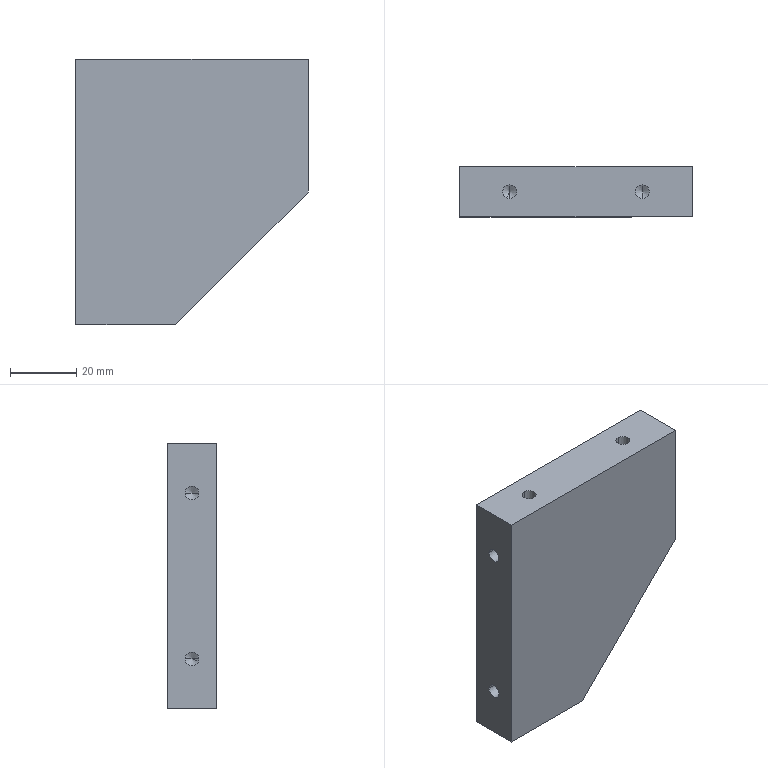Component | SolidWorks | BeveledAluminumSupport-1 | 1 solid | 23 faces | box 70 x 15 x 80 mm | volume 71290 mm3 | cylinder 8 | cone 8 | plane 7 | commonest cylinder face diameters 4.2 x8
build123d program:
from build123d import *

# Parameters (mm, degrees)
BOSS_EXTRUDE1_DEPTH   = 7.5
M5_TAPPED_HOLE1_D     = 4.2
M5_TAPPED_HOLE1_DEPTH = 12.4
M5_TAPPED_HOLE1_TIP   = 1.212
M5_TAPPED_HOLE2_D     = 4.2
M5_TAPPED_HOLE2_DEPTH = 12.4
M5_TAPPED_HOLE2_TIP   = 1.212


with BuildPart() as part:
    # Sketch1 → Boss-Extrude1 (new, symmetric)
    with BuildSketch(Plane.XY):
        Polygon((30, 80), (70, 40), (70, 0), (0, 0), (0, 80), align=None)
    extrude(amount=BOSS_EXTRUDE1_DEPTH, both=True)

    # M5 Tapped Hole1
    with Locations(Plane(origin=(0, 65, 0), x_dir=(0, 0, -1), z_dir=(-1, 0, 0))):
        with Locations((0, 0), (0, 50)):
            Hole(M5_TAPPED_HOLE1_D / 2, depth=M5_TAPPED_HOLE1_DEPTH)
            with Locations((0, 0, -(M5_TAPPED_HOLE1_DEPTH + M5_TAPPED_HOLE1_TIP / 2))):  # 120° drill point
                Cone(0, M5_TAPPED_HOLE1_D / 2, M5_TAPPED_HOLE1_TIP, mode=Mode.SUBTRACT)

    # M5 Tapped Hole2
    with Locations(Plane(origin=(15, 0, 0), x_dir=(0, 0, -1), z_dir=(0, -1, 0))):
        with Locations((0, 0), (0, 40)):
            Hole(M5_TAPPED_HOLE2_D / 2, depth=M5_TAPPED_HOLE2_DEPTH)
            with Locations((0, 0, -(M5_TAPPED_HOLE2_DEPTH + M5_TAPPED_HOLE2_TIP / 2))):  # 120° drill point
                Cone(0, M5_TAPPED_HOLE2_D / 2, M5_TAPPED_HOLE2_TIP, mode=Mode.SUBTRACT)


solid = part.part

# Placed as in the assembly
solid = solid.moved(Location((2.915, 37.185, 71.225), (-90, 0, 0)))
STEP:
#1=COLOUR_RGB('',0.7922,0.8196,0.9333);
#2=FILL_AREA_STYLE_COLOUR('',#1);
#3=FILL_AREA_STYLE('',(#2));
#4=SURFACE_STYLE_FILL_AREA(#3);
#5=SURFACE_SIDE_STYLE('',(#4));
#6=SURFACE_STYLE_USAGE(.BOTH.,#5);
#7=PRESENTATION_STYLE_ASSIGNMENT((#6));
#8=CARTESIAN_POINT('',(0.7053,1.547,2.316));
#9=VERTEX_POINT('',#8);
#10=CARTESIAN_POINT('',(0.7053,1.381,2.316));
#11=VERTEX_POINT('',#10);
#12=CARTESIAN_POINT('',(0.7053,1.464,2.316));
#13=DIRECTION('',(0.,0.,1.));
#14=DIRECTION('',(0.,-1.,0.));
#15=AXIS2_PLACEMENT_3D('',#12,#13,#14);
#16=CIRCLE('',#15,0.08268);
#17=EDGE_CURVE('',#9,#11,#16,.T.);
#18=ORIENTED_EDGE('',*,*,#17,.F.);
#19=CARTESIAN_POINT('',(0.7053,1.547,2.804));
#20=VERTEX_POINT('',#19);
#21=CARTESIAN_POINT('',(0.7053,1.547,2.804));
#22=DIRECTION('',(0.,0.,1.));
#23=VECTOR('',#22,39.37);
#24=LINE('',#21,#23);
#25=EDGE_CURVE('',#9,#20,#24,.T.);
#26=ORIENTED_EDGE('',*,*,#25,.T.);
#27=CARTESIAN_POINT('',(0.7053,1.381,2.804));
#28=VERTEX_POINT('',#27);
#29=CARTESIAN_POINT('',(0.7053,1.464,2.804));
#30=DIRECTION('',(0.,0.,1.));
#31=DIRECTION('',(0.,-1.,0.));
#32=AXIS2_PLACEMENT_3D('',#29,#30,#31);
#33=CIRCLE('',#32,0.08268);
#34=EDGE_CURVE('',#20,#28,#33,.T.);
#35=ORIENTED_EDGE('',*,*,#34,.T.);
#36=CARTESIAN_POINT('',(0.7053,1.381,2.804));
#37=DIRECTION('',(0.,0.,1.));
#38=VECTOR('',#37,39.37);
#39=LINE('',#36,#38);
#40=EDGE_CURVE('',#11,#28,#39,.T.);
#41=ORIENTED_EDGE('',*,*,#40,.F.);
#42=EDGE_LOOP('',(#18,#26,#35,#41));
#43=FACE_OUTER_BOUND('',#42,.T.);
#44=CARTESIAN_POINT('',(0.7053,1.464,2.804));
#45=DIRECTION('',(0.,0.,1.));
#46=DIRECTION('',(0.,-1.,0.));
#47=AXIS2_PLACEMENT_3D('',#44,#45,#46);
#48=CYLINDRICAL_SURFACE('',#47,0.08268);
#49=ADVANCED_FACE('',(#43),#48,.F.);
#50=CARTESIAN_POINT('',(0.7053,1.464,2.268));
#51=VERTEX_POINT('',#50);
#52=CARTESIAN_POINT('',(0.7053,1.381,2.316));
#53=DIRECTION('',(0.,-0.866,0.5));
#54=VECTOR('',#53,39.37);
#55=LINE('',#52,#54);
#56=EDGE_CURVE('',#51,#11,#55,.T.);
#57=ORIENTED_EDGE('',*,*,#56,.F.);
#58=CARTESIAN_POINT('',(0.7053,1.547,2.316));
#59=DIRECTION('',(0.,0.866,0.5));
#60=VECTOR('',#59,39.37);
#61=LINE('',#58,#60);
#62=EDGE_CURVE('',#51,#9,#61,.T.);
#63=ORIENTED_EDGE('',*,*,#62,.T.);
#64=ORIENTED_EDGE('',*,*,#17,.T.);
#65=EDGE_LOOP('',(#57,#63,#64));
#66=FACE_OUTER_BOUND('',#65,.T.);
#67=CARTESIAN_POINT('',(0.7053,1.464,2.316));
#68=DIRECTION('',(0.,0.,1.));
#69=DIRECTION('',(0.,-1.,0.));
#70=AXIS2_PLACEMENT_3D('',#67,#68,#69);
#71=CONICAL_SURFACE('',#70,0.08268,1.047);
#72=ADVANCED_FACE('',(#66),#71,.F.);
#73=CARTESIAN_POINT('',(2.28,1.547,2.316));
#74=VERTEX_POINT('',#73);
#75=CARTESIAN_POINT('',(2.28,1.381,2.316));
#76=VERTEX_POINT('',#75);
#77=CARTESIAN_POINT('',(2.28,1.464,2.316));
#78=DIRECTION('',(0.,0.,1.));
#79=DIRECTION('',(0.,-1.,0.));
#80=AXIS2_PLACEMENT_3D('',#77,#78,#79);
#81=CIRCLE('',#80,0.08268);
#82=EDGE_CURVE('',#74,#76,#81,.T.);
#83=ORIENTED_EDGE('',*,*,#82,.F.);
#84=CARTESIAN_POINT('',(2.28,1.547,2.804));
#85=VERTEX_POINT('',#84);
#86=CARTESIAN_POINT('',(2.28,1.547,2.804));
#87=DIRECTION('',(0.,0.,1.));
#88=VECTOR('',#87,39.37);
#89=LINE('',#86,#88);
#90=EDGE_CURVE('',#74,#85,#89,.T.);
#91=ORIENTED_EDGE('',*,*,#90,.T.);
#92=CARTESIAN_POINT('',(2.28,1.381,2.804));
#93=VERTEX_POINT('',#92);
#94=CARTESIAN_POINT('',(2.28,1.464,2.804));
#95=DIRECTION('',(0.,0.,1.));
#96=DIRECTION('',(0.,-1.,0.));
#97=AXIS2_PLACEMENT_3D('',#94,#95,#96);
#98=CIRCLE('',#97,0.08268);
#99=EDGE_CURVE('',#85,#93,#98,.T.);
#100=ORIENTED_EDGE('',*,*,#99,.T.);
#101=CARTESIAN_POINT('',(2.28,1.381,2.804));
#102=DIRECTION('',(0.,0.,1.));
#103=VECTOR('',#102,39.37);
#104=LINE('',#101,#103);
#105=EDGE_CURVE('',#76,#93,#104,.T.);
#106=ORIENTED_EDGE('',*,*,#105,.F.);
#107=EDGE_LOOP('',(#83,#91,#100,#106));
#108=FACE_OUTER_BOUND('',#107,.T.);
#109=CARTESIAN_POINT('',(2.28,1.464,2.804));
#110=DIRECTION('',(0.,0.,1.));
#111=DIRECTION('',(0.,-1.,0.));
#112=AXIS2_PLACEMENT_3D('',#109,#110,#111);
#113=CYLINDRICAL_SURFACE('',#112,0.08268);
#114=ADVANCED_FACE('',(#108),#113,.F.);
#115=CARTESIAN_POINT('',(2.28,1.464,2.268));
#116=VERTEX_POINT('',#115);
#117=CARTESIAN_POINT('',(2.28,1.381,2.316));
#118=DIRECTION('',(0.,-0.866,0.5));
#119=VECTOR('',#118,39.37);
#120=LINE('',#117,#119);
#121=EDGE_CURVE('',#116,#76,#120,.T.);
#122=ORIENTED_EDGE('',*,*,#121,.F.);
#123=CARTESIAN_POINT('',(2.28,1.547,2.316));
#124=DIRECTION('',(0.,0.866,0.5));
#125=VECTOR('',#124,39.37);
#126=LINE('',#123,#125);
#127=EDGE_CURVE('',#116,#74,#126,.T.);
#128=ORIENTED_EDGE('',*,*,#127,.T.);
#129=ORIENTED_EDGE('',*,*,#82,.T.);
#130=EDGE_LOOP('',(#122,#128,#129));
#131=FACE_OUTER_BOUND('',#130,.T.);
#132=CARTESIAN_POINT('',(2.28,1.464,2.316));
#133=DIRECTION('',(0.,0.,1.));
#134=DIRECTION('',(0.,-1.,0.));
#135=AXIS2_PLACEMENT_3D('',#132,#133,#134);
#136=CONICAL_SURFACE('',#135,0.08268,1.047);
#137=ADVANCED_FACE('',(#131),#136,.F.);
#138=CARTESIAN_POINT('',(0.603,1.381,0.2451));
#139=VERTEX_POINT('',#138);
#140=CARTESIAN_POINT('',(0.603,1.547,0.2451));
#141=VERTEX_POINT('',#140);
#142=CARTESIAN_POINT('',(0.603,1.464,0.2451));
#143=DIRECTION('',(-1.,0.,0.));
#144=DIRECTION('',(0.,1.,0.));
#145=AXIS2_PLACEMENT_3D('',#142,#143,#144);
#146=CIRCLE('',#145,0.08268);
#147=EDGE_CURVE('',#139,#141,#146,.T.);
#148=ORIENTED_EDGE('',*,*,#147,.F.);
#149=CARTESIAN_POINT('',(0.1148,1.381,0.2451));
#150=VERTEX_POINT('',#149);
#151=CARTESIAN_POINT('',(0.1148,1.381,0.2451));
#152=DIRECTION('',(-1.,0.,0.));
#153=VECTOR('',#152,39.37);
#154=LINE('',#151,#153);
#155=EDGE_CURVE('',#139,#150,#154,.T.);
#156=ORIENTED_EDGE('',*,*,#155,.T.);
#157=CARTESIAN_POINT('',(0.1148,1.547,0.2451));
#158=VERTEX_POINT('',#157);
#159=CARTESIAN_POINT('',(0.1148,1.464,0.2451));
#160=DIRECTION('',(-1.,0.,0.));
#161=DIRECTION('',(0.,1.,0.));
#162=AXIS2_PLACEMENT_3D('',#159,#160,#161);
#163=CIRCLE('',#162,0.08268);
#164=EDGE_CURVE('',#150,#158,#163,.T.);
#165=ORIENTED_EDGE('',*,*,#164,.T.);
#166=CARTESIAN_POINT('',(0.1148,1.547,0.2451));
#167=DIRECTION('',(-1.,0.,0.));
#168=VECTOR('',#167,39.37);
#169=LINE('',#166,#168);
#170=EDGE_CURVE('',#141,#158,#169,.T.);
#171=ORIENTED_EDGE('',*,*,#170,.F.);
#172=EDGE_LOOP('',(#148,#156,#165,#171));
#173=FACE_OUTER_BOUND('',#172,.T.);
#174=CARTESIAN_POINT('',(0.1148,1.464,0.2451));
#175=DIRECTION('',(-1.,0.,0.));
#176=DIRECTION('',(0.,1.,0.));
#177=AXIS2_PLACEMENT_3D('',#174,#175,#176);
#178=CYLINDRICAL_SURFACE('',#177,0.08268);
#179=ADVANCED_FACE('',(#173),#178,.F.);
#180=CARTESIAN_POINT('',(0.6507,1.464,0.2451));
#181=VERTEX_POINT('',#180);
#182=CARTESIAN_POINT('',(0.603,1.547,0.2451));
#183=DIRECTION('',(-0.5,0.866,0.));
#184=VECTOR('',#183,39.37);
#185=LINE('',#182,#184);
#186=EDGE_CURVE('',#181,#141,#185,.T.);
#187=ORIENTED_EDGE('',*,*,#186,.F.);
#188=CARTESIAN_POINT('',(0.603,1.381,0.2451));
#189=DIRECTION('',(-0.5,-0.866,-0.));
#190=VECTOR('',#189,39.37);
#191=LINE('',#188,#190);
#192=EDGE_CURVE('',#181,#139,#191,.T.);
#193=ORIENTED_EDGE('',*,*,#192,.T.);
#194=ORIENTED_EDGE('',*,*,#147,.T.);
#195=EDGE_LOOP('',(#187,#193,#194));
#196=FACE_OUTER_BOUND('',#195,.T.);
#197=CARTESIAN_POINT('',(0.603,1.464,0.2451));
#198=DIRECTION('',(-1.,0.,0.));
#199=DIRECTION('',(0.,1.,0.));
#200=AXIS2_PLACEMENT_3D('',#197,#198,#199);
#201=CONICAL_SURFACE('',#200,0.08268,1.047);
#202=ADVANCED_FACE('',(#196),#201,.F.);
#203=CARTESIAN_POINT('',(0.603,1.381,2.214));
#204=VERTEX_POINT('',#203);
#205=CARTESIAN_POINT('',(0.603,1.547,2.214));
#206=VERTEX_POINT('',#205);
#207=CARTESIAN_POINT('',(0.603,1.464,2.214));
#208=DIRECTION('',(-1.,0.,0.));
#209=DIRECTION('',(0.,1.,0.));
#210=AXIS2_PLACEMENT_3D('',#207,#208,#209);
#211=CIRCLE('',#210,0.08268);
#212=EDGE_CURVE('',#204,#206,#211,.T.);
#213=ORIENTED_EDGE('',*,*,#212,.F.);
#214=CARTESIAN_POINT('',(0.1148,1.381,2.214));
#215=VERTEX_POINT('',#214);
#216=CARTESIAN_POINT('',(0.1148,1.381,2.214));
#217=DIRECTION('',(-1.,0.,0.));
#218=VECTOR('',#217,39.37);
#219=LINE('',#216,#218);
#220=EDGE_CURVE('',#204,#215,#219,.T.);
#221=ORIENTED_EDGE('',*,*,#220,.T.);
#222=CARTESIAN_POINT('',(0.1148,1.547,2.214));
#223=VERTEX_POINT('',#222);
#224=CARTESIAN_POINT('',(0.1148,1.464,2.214));
#225=DIRECTION('',(-1.,0.,0.));
#226=DIRECTION('',(0.,1.,0.));
#227=AXIS2_PLACEMENT_3D('',#224,#225,#226);
#228=CIRCLE('',#227,0.08268);
#229=EDGE_CURVE('',#215,#223,#228,.T.);
#230=ORIENTED_EDGE('',*,*,#229,.T.);
#231=CARTESIAN_POINT('',(0.1148,1.547,2.214));
#232=DIRECTION('',(-1.,0.,0.));
#233=VECTOR('',#232,39.37);
#234=LINE('',#231,#233);
#235=EDGE_CURVE('',#206,#223,#234,.T.);
#236=ORIENTED_EDGE('',*,*,#235,.F.);
#237=EDGE_LOOP('',(#213,#221,#230,#236));
#238=FACE_OUTER_BOUND('',#237,.T.);
#239=CARTESIAN_POINT('',(0.1148,1.464,2.214));
#240=DIRECTION('',(-1.,0.,0.));
#241=DIRECTION('',(0.,1.,0.));
#242=AXIS2_PLACEMENT_3D('',#239,#240,#241);
#243=CYLINDRICAL_SURFACE('',#242,0.08268);
#244=ADVANCED_FACE('',(#238),#243,.F.);
#245=CARTESIAN_POINT('',(0.6507,1.464,2.214));
#246=VERTEX_POINT('',#245);
#247=CARTESIAN_POINT('',(0.603,1.547,2.214));
#248=DIRECTION('',(-0.5,0.866,0.));
#249=VECTOR('',#248,39.37);
#250=LINE('',#247,#249);
#251=EDGE_CURVE('',#246,#206,#250,.T.);
#252=ORIENTED_EDGE('',*,*,#251,.F.);
#253=CARTESIAN_POINT('',(0.603,1.381,2.214));
#254=DIRECTION('',(-0.5,-0.866,-0.));
#255=VECTOR('',#254,39.37);
#256=LINE('',#253,#255);
#257=EDGE_CURVE('',#246,#204,#256,.T.);
#258=ORIENTED_EDGE('',*,*,#257,.T.);
#259=ORIENTED_EDGE('',*,*,#212,.T.);
#260=EDGE_LOOP('',(#252,#258,#259));
#261=FACE_OUTER_BOUND('',#260,.T.);
#262=CARTESIAN_POINT('',(0.603,1.464,2.214));
#263=DIRECTION('',(-1.,0.,0.));
#264=DIRECTION('',(0.,1.,0.));
#265=AXIS2_PLACEMENT_3D('',#262,#263,#264);
#266=CONICAL_SURFACE('',#265,0.08268,1.047);
#267=ADVANCED_FACE('',(#261),#266,.F.);
#268=CARTESIAN_POINT('',(0.1148,1.464,0.2451));
#269=DIRECTION('',(-1.,0.,0.));
#270=DIRECTION('',(0.,1.,0.));
#271=AXIS2_PLACEMENT_3D('',#268,#269,#270);
#272=CIRCLE('',#271,0.08268);
#273=EDGE_CURVE('',#158,#150,#272,.T.);
#274=ORIENTED_EDGE('',*,*,#273,.F.);
#275=ORIENTED_EDGE('',*,*,#164,.F.);
#276=EDGE_LOOP('',(#274,#275));
#277=FACE_BOUND('',#276,.T.);
#278=CARTESIAN_POINT('',(0.1148,1.464,2.214));
#279=DIRECTION('',(-1.,0.,0.));
#280=DIRECTION('',(0.,1.,0.));
#281=AXIS2_PLACEMENT_3D('',#278,#279,#280);
#282=CIRCLE('',#281,0.08268);
#283=EDGE_CURVE('',#223,#215,#282,.T.);
#284=ORIENTED_EDGE('',*,*,#283,.F.);
#285=ORIENTED_EDGE('',*,*,#229,.F.);
#286=EDGE_LOOP('',(#284,#285));
#287=FACE_BOUND('',#286,.T.);
#288=CARTESIAN_POINT('',(0.1148,1.169,-0.3455));
#289=VERTEX_POINT('',#288);
#290=CARTESIAN_POINT('',(0.1148,1.169,2.804));
#291=VERTEX_POINT('',#290);
#292=CARTESIAN_POINT('',(0.1148,1.169,2.804));
#293=DIRECTION('',(0.,0.,1.));
#294=VECTOR('',#293,39.37);
#295=LINE('',#292,#294);
#296=EDGE_CURVE('',#289,#291,#295,.T.);
#297=ORIENTED_EDGE('',*,*,#296,.T.);
#298=CARTESIAN_POINT('',(0.1148,1.759,2.804));
#299=VERTEX_POINT('',#298);
#300=CARTESIAN_POINT('',(0.1148,1.759,2.804));
#301=DIRECTION('',(0.,-1.,0.));
#302=VECTOR('',#301,39.37);
#303=LINE('',#300,#302);
#304=EDGE_CURVE('',#299,#291,#303,.T.);
#305=ORIENTED_EDGE('',*,*,#304,.F.);
#306=CARTESIAN_POINT('',(0.1148,1.759,-0.3455));
#307=VERTEX_POINT('',#306);
#308=CARTESIAN_POINT('',(0.1148,1.759,2.804));
#309=DIRECTION('',(0.,0.,1.));
#310=VECTOR('',#309,39.37);
#311=LINE('',#308,#310);
#312=EDGE_CURVE('',#307,#299,#311,.T.);
#313=ORIENTED_EDGE('',*,*,#312,.F.);
#314=CARTESIAN_POINT('',(0.1148,1.759,-0.3455));
#315=DIRECTION('',(0.,-1.,0.));
#316=VECTOR('',#315,39.37);
#317=LINE('',#314,#316);
#318=EDGE_CURVE('',#307,#289,#317,.T.);
#319=ORIENTED_EDGE('',*,*,#318,.T.);
#320=EDGE_LOOP('',(#297,#305,#313,#319));
#321=FACE_OUTER_BOUND('',#320,.T.);
#322=CARTESIAN_POINT('',(0.1148,1.759,2.804));
#323=DIRECTION('',(1.,-0.,-0.));
#324=DIRECTION('',(0.,-1.,0.));
#325=AXIS2_PLACEMENT_3D('',#322,#323,#324);
#326=PLANE('',#325);
#327=ADVANCED_FACE('',(#277,#287,#321),#326,.F.);
#328=CARTESIAN_POINT('',(0.7053,1.464,2.804));
#329=DIRECTION('',(0.,0.,1.));
#330=DIRECTION('',(0.,-1.,0.));
#331=AXIS2_PLACEMENT_3D('',#328,#329,#330);
#332=CIRCLE('',#331,0.08268);
#333=EDGE_CURVE('',#28,#20,#332,.T.);
#334=ORIENTED_EDGE('',*,*,#333,.F.);
#335=ORIENTED_EDGE('',*,*,#34,.F.);
#336=EDGE_LOOP('',(#334,#335));
#337=FACE_BOUND('',#336,.T.);
#338=CARTESIAN_POINT('',(2.28,1.464,2.804));
#339=DIRECTION('',(0.,0.,1.));
#340=DIRECTION('',(0.,-1.,0.));
#341=AXIS2_PLACEMENT_3D('',#338,#339,#340);
#342=CIRCLE('',#341,0.08268);
#343=EDGE_CURVE('',#93,#85,#342,.T.);
#344=ORIENTED_EDGE('',*,*,#343,.F.);
#345=ORIENTED_EDGE('',*,*,#99,.F.);
#346=EDGE_LOOP('',(#344,#345));
#347=FACE_BOUND('',#346,.T.);
#348=CARTESIAN_POINT('',(2.871,1.169,2.804));
#349=VERTEX_POINT('',#348);
#350=CARTESIAN_POINT('',(0.1148,1.169,2.804));
#351=DIRECTION('',(1.,0.,-0.));
#352=VECTOR('',#351,39.37);
#353=LINE('',#350,#352);
#354=EDGE_CURVE('',#291,#349,#353,.T.);
#355=ORIENTED_EDGE('',*,*,#354,.T.);
#356=CARTESIAN_POINT('',(2.871,1.759,2.804));
#357=VERTEX_POINT('',#356);
#358=CARTESIAN_POINT('',(2.871,1.759,2.804));
#359=DIRECTION('',(0.,-1.,0.));
#360=VECTOR('',#359,39.37);
#361=LINE('',#358,#360);
#362=EDGE_CURVE('',#357,#349,#361,.T.);
#363=ORIENTED_EDGE('',*,*,#362,.F.);
#364=CARTESIAN_POINT('',(0.1148,1.759,2.804));
#365=DIRECTION('',(1.,0.,-0.));
#366=VECTOR('',#365,39.37);
#367=LINE('',#364,#366);
#368=EDGE_CURVE('',#299,#357,#367,.T.);
#369=ORIENTED_EDGE('',*,*,#368,.F.);
#370=ORIENTED_EDGE('',*,*,#304,.T.);
#371=EDGE_LOOP('',(#355,#363,#369,#370));
#372=FACE_OUTER_BOUND('',#371,.T.);
#373=CARTESIAN_POINT('',(0.1148,1.759,2.804));
#374=DIRECTION('',(-0.,-0.,-1.));
#375=DIRECTION('',(0.,1.,-0.));
#376=AXIS2_PLACEMENT_3D('',#373,#374,#375);
#377=PLANE('',#376);
#378=ADVANCED_FACE('',(#337,#347,#372),#377,.F.);
#379=CARTESIAN_POINT('',(2.871,1.169,1.229));
#380=VERTEX_POINT('',#379);
#381=CARTESIAN_POINT('',(2.871,1.169,2.804));
#382=DIRECTION('',(-0.,-0.,-1.));
#383=VECTOR('',#382,39.37);
#384=LINE('',#381,#383);
#385=EDGE_CURVE('',#349,#380,#384,.T.);
#386=ORIENTED_EDGE('',*,*,#385,.T.);
#387=CARTESIAN_POINT('',(2.871,1.759,1.229));
#388=VERTEX_POINT('',#387);
#389=CARTESIAN_POINT('',(2.871,1.759,1.229));
#390=DIRECTION('',(0.,-1.,0.));
#391=VECTOR('',#390,39.37);
#392=LINE('',#389,#391);
#393=EDGE_CURVE('',#388,#380,#392,.T.);
#394=ORIENTED_EDGE('',*,*,#393,.F.);
#395=CARTESIAN_POINT('',(2.871,1.759,2.804));
#396=DIRECTION('',(-0.,-0.,-1.));
#397=VECTOR('',#396,39.37);
#398=LINE('',#395,#397);
#399=EDGE_CURVE('',#357,#388,#398,.T.);
#400=ORIENTED_EDGE('',*,*,#399,.F.);
#401=ORIENTED_EDGE('',*,*,#362,.T.);
#402=EDGE_LOOP('',(#386,#394,#400,#401));
#403=FACE_OUTER_BOUND('',#402,.T.);
#404=CARTESIAN_POINT('',(2.871,1.759,2.804));
#405=DIRECTION('',(-1.,0.,0.));
#406=DIRECTION('',(0.,1.,-0.));
#407=AXIS2_PLACEMENT_3D('',#404,#405,#406);
#408=PLANE('',#407);
#409=ADVANCED_FACE('',(#403),#408,.F.);
#410=CARTESIAN_POINT('',(1.296,1.169,-0.3455));
#411=VERTEX_POINT('',#410);
#412=CARTESIAN_POINT('',(1.296,1.169,-0.3455));
#413=DIRECTION('',(-0.7071,-0.,-0.7071));
#414=VECTOR('',#413,39.37);
#415=LINE('',#412,#414);
#416=EDGE_CURVE('',#380,#411,#415,.T.);
#417=ORIENTED_EDGE('',*,*,#416,.T.);
#418=CARTESIAN_POINT('',(1.296,1.759,-0.3455));
#419=VERTEX_POINT('',#418);
#420=CARTESIAN_POINT('',(1.296,1.759,-0.3455));
#421=DIRECTION('',(0.,-1.,0.));
#422=VECTOR('',#421,39.37);
#423=LINE('',#420,#422);
#424=EDGE_CURVE('',#419,#411,#423,.T.);
#425=ORIENTED_EDGE('',*,*,#424,.F.);
#426=CARTESIAN_POINT('',(1.296,1.759,-0.3455));
#427=DIRECTION('',(-0.7071,-0.,-0.7071));
#428=VECTOR('',#427,39.37);
#429=LINE('',#426,#428);
#430=EDGE_CURVE('',#388,#419,#429,.T.);
#431=ORIENTED_EDGE('',*,*,#430,.F.);
#432=ORIENTED_EDGE('',*,*,#393,.T.);
#433=EDGE_LOOP('',(#417,#425,#431,#432));
#434=FACE_OUTER_BOUND('',#433,.T.);
#435=CARTESIAN_POINT('',(1.296,1.759,-0.3455));
#436=DIRECTION('',(-0.7071,0.,0.7071));
#437=DIRECTION('',(0.7071,0.,0.7071));
#438=AXIS2_PLACEMENT_3D('',#435,#436,#437);
#439=PLANE('',#438);
#440=ADVANCED_FACE('',(#434),#439,.F.);
#441=CARTESIAN_POINT('',(0.1148,1.169,-0.3455));
#442=DIRECTION('',(-1.,0.,0.));
#443=VECTOR('',#442,39.37);
#444=LINE('',#441,#443);
#445=EDGE_CURVE('',#411,#289,#444,.T.);
#446=ORIENTED_EDGE('',*,*,#445,.T.);
#447=ORIENTED_EDGE('',*,*,#318,.F.);
#448=CARTESIAN_POINT('',(0.1148,1.759,-0.3455));
#449=DIRECTION('',(-1.,0.,0.));
#450=VECTOR('',#449,39.37);
#451=LINE('',#448,#450);
#452=EDGE_CURVE('',#419,#307,#451,.T.);
#453=ORIENTED_EDGE('',*,*,#452,.F.);
#454=ORIENTED_EDGE('',*,*,#424,.T.);
#455=EDGE_LOOP('',(#446,#447,#453,#454));
#456=FACE_OUTER_BOUND('',#455,.T.);
#457=CARTESIAN_POINT('',(0.1148,1.759,-0.3455));
#458=DIRECTION('',(0.,0.,1.));
#459=DIRECTION('',(0.,-1.,0.));
#460=AXIS2_PLACEMENT_3D('',#457,#458,#459);
#461=PLANE('',#460);
#462=ADVANCED_FACE('',(#456),#461,.F.);
#463=ORIENTED_EDGE('',*,*,#312,.T.);
#464=ORIENTED_EDGE('',*,*,#368,.T.);
#465=ORIENTED_EDGE('',*,*,#399,.T.);
#466=ORIENTED_EDGE('',*,*,#430,.T.);
#467=ORIENTED_EDGE('',*,*,#452,.T.);
#468=EDGE_LOOP('',(#463,#464,#465,#466,#467));
#469=FACE_OUTER_BOUND('',#468,.T.);
#470=CARTESIAN_POINT('',(0.1148,1.759,2.804));
#471=DIRECTION('',(0.,-1.,0.));
#472=DIRECTION('',(-1.,0.,0.));
#473=AXIS2_PLACEMENT_3D('',#470,#471,#472);
#474=PLANE('',#473);
#475=ADVANCED_FACE('',(#469),#474,.F.);
#476=ORIENTED_EDGE('',*,*,#296,.F.);
#477=ORIENTED_EDGE('',*,*,#445,.F.);
#478=ORIENTED_EDGE('',*,*,#416,.F.);
#479=ORIENTED_EDGE('',*,*,#385,.F.);
#480=ORIENTED_EDGE('',*,*,#354,.F.);
#481=EDGE_LOOP('',(#476,#477,#478,#479,#480));
#482=FACE_OUTER_BOUND('',#481,.T.);
#483=CARTESIAN_POINT('',(0.1148,1.169,2.804));
#484=DIRECTION('',(0.,-1.,0.));
#485=DIRECTION('',(-1.,0.,0.));
#486=AXIS2_PLACEMENT_3D('',#483,#484,#485);
#487=PLANE('',#486);
#488=ADVANCED_FACE('',(#482),#487,.T.);
#489=ORIENTED_EDGE('',*,*,#257,.F.);
#490=ORIENTED_EDGE('',*,*,#251,.T.);
#491=CARTESIAN_POINT('',(0.603,1.464,2.214));
#492=DIRECTION('',(-1.,0.,0.));
#493=DIRECTION('',(0.,1.,0.));
#494=AXIS2_PLACEMENT_3D('',#491,#492,#493);
#495=CIRCLE('',#494,0.08268);
#496=EDGE_CURVE('',#206,#204,#495,.T.);
#497=ORIENTED_EDGE('',*,*,#496,.T.);
#498=EDGE_LOOP('',(#489,#490,#497));
#499=FACE_OUTER_BOUND('',#498,.T.);
#500=CARTESIAN_POINT('',(0.603,1.464,2.214));
#501=DIRECTION('',(-1.,0.,0.));
#502=DIRECTION('',(0.,1.,0.));
#503=AXIS2_PLACEMENT_3D('',#500,#501,#502);
#504=CONICAL_SURFACE('',#503,0.08268,1.047);
#505=ADVANCED_FACE('',(#499),#504,.F.);
#506=ORIENTED_EDGE('',*,*,#220,.F.);
#507=ORIENTED_EDGE('',*,*,#496,.F.);
#508=ORIENTED_EDGE('',*,*,#235,.T.);
#509=ORIENTED_EDGE('',*,*,#283,.T.);
#510=EDGE_LOOP('',(#506,#507,#508,#509));
#511=FACE_OUTER_BOUND('',#510,.T.);
#512=CARTESIAN_POINT('',(0.1148,1.464,2.214));
#513=DIRECTION('',(-1.,0.,0.));
#514=DIRECTION('',(0.,1.,0.));
#515=AXIS2_PLACEMENT_3D('',#512,#513,#514);
#516=CYLINDRICAL_SURFACE('',#515,0.08268);
#517=ADVANCED_FACE('',(#511),#516,.F.);
#518=ORIENTED_EDGE('',*,*,#192,.F.);
#519=ORIENTED_EDGE('',*,*,#186,.T.);
#520=CARTESIAN_POINT('',(0.603,1.464,0.2451));
#521=DIRECTION('',(-1.,0.,0.));
#522=DIRECTION('',(0.,1.,0.));
#523=AXIS2_PLACEMENT_3D('',#520,#521,#522);
#524=CIRCLE('',#523,0.08268);
#525=EDGE_CURVE('',#141,#139,#524,.T.);
#526=ORIENTED_EDGE('',*,*,#525,.T.);
#527=EDGE_LOOP('',(#518,#519,#526));
#528=FACE_OUTER_BOUND('',#527,.T.);
#529=CARTESIAN_POINT('',(0.603,1.464,0.2451));
#530=DIRECTION('',(-1.,0.,0.));
#531=DIRECTION('',(0.,1.,0.));
#532=AXIS2_PLACEMENT_3D('',#529,#530,#531);
#533=CONICAL_SURFACE('',#532,0.08268,1.047);
#534=ADVANCED_FACE('',(#528),#533,.F.);
#535=ORIENTED_EDGE('',*,*,#155,.F.);
#536=ORIENTED_EDGE('',*,*,#525,.F.);
#537=ORIENTED_EDGE('',*,*,#170,.T.);
#538=ORIENTED_EDGE('',*,*,#273,.T.);
#539=EDGE_LOOP('',(#535,#536,#537,#538));
#540=FACE_OUTER_BOUND('',#539,.T.);
#541=CARTESIAN_POINT('',(0.1148,1.464,0.2451));
#542=DIRECTION('',(-1.,0.,0.));
#543=DIRECTION('',(0.,1.,0.));
#544=AXIS2_PLACEMENT_3D('',#541,#542,#543);
#545=CYLINDRICAL_SURFACE('',#544,0.08268);
#546=ADVANCED_FACE('',(#540),#545,.F.);
#547=ORIENTED_EDGE('',*,*,#127,.F.);
#548=ORIENTED_EDGE('',*,*,#121,.T.);
#549=CARTESIAN_POINT('',(2.28,1.464,2.316));
#550=DIRECTION('',(0.,0.,1.));
#551=DIRECTION('',(0.,-1.,0.));
#552=AXIS2_PLACEMENT_3D('',#549,#550,#551);
#553=CIRCLE('',#552,0.08268);
#554=EDGE_CURVE('',#76,#74,#553,.T.);
#555=ORIENTED_EDGE('',*,*,#554,.T.);
#556=EDGE_LOOP('',(#547,#548,#555));
#557=FACE_OUTER_BOUND('',#556,.T.);
#558=CARTESIAN_POINT('',(2.28,1.464,2.316));
#559=DIRECTION('',(0.,0.,1.));
#560=DIRECTION('',(0.,-1.,0.));
#561=AXIS2_PLACEMENT_3D('',#558,#559,#560);
#562=CONICAL_SURFACE('',#561,0.08268,1.047);
#563=ADVANCED_FACE('',(#557),#562,.F.);
#564=ORIENTED_EDGE('',*,*,#90,.F.);
#565=ORIENTED_EDGE('',*,*,#554,.F.);
#566=ORIENTED_EDGE('',*,*,#105,.T.);
#567=ORIENTED_EDGE('',*,*,#343,.T.);
#568=EDGE_LOOP('',(#564,#565,#566,#567));
#569=FACE_OUTER_BOUND('',#568,.T.);
#570=CARTESIAN_POINT('',(2.28,1.464,2.804));
#571=DIRECTION('',(0.,0.,1.));
#572=DIRECTION('',(0.,-1.,0.));
#573=AXIS2_PLACEMENT_3D('',#570,#571,#572);
#574=CYLINDRICAL_SURFACE('',#573,0.08268);
#575=ADVANCED_FACE('',(#569),#574,.F.);
#576=ORIENTED_EDGE('',*,*,#62,.F.);
#577=ORIENTED_EDGE('',*,*,#56,.T.);
#578=CARTESIAN_POINT('',(0.7053,1.464,2.316));
#579=DIRECTION('',(0.,0.,1.));
#580=DIRECTION('',(0.,-1.,0.));
#581=AXIS2_PLACEMENT_3D('',#578,#579,#580);
#582=CIRCLE('',#581,0.08268);
#583=EDGE_CURVE('',#11,#9,#582,.T.);
#584=ORIENTED_EDGE('',*,*,#583,.T.);
#585=EDGE_LOOP('',(#576,#577,#584));
#586=FACE_OUTER_BOUND('',#585,.T.);
#587=CARTESIAN_POINT('',(0.7053,1.464,2.316));
#588=DIRECTION('',(0.,0.,1.));
#589=DIRECTION('',(0.,-1.,0.));
#590=AXIS2_PLACEMENT_3D('',#587,#588,#589);
#591=CONICAL_SURFACE('',#590,0.08268,1.047);
#592=ADVANCED_FACE('',(#586),#591,.F.);
#593=ORIENTED_EDGE('',*,*,#25,.F.);
#594=ORIENTED_EDGE('',*,*,#583,.F.);
#595=ORIENTED_EDGE('',*,*,#40,.T.);
#596=ORIENTED_EDGE('',*,*,#333,.T.);
#597=EDGE_LOOP('',(#593,#594,#595,#596));
#598=FACE_OUTER_BOUND('',#597,.T.);
#599=CARTESIAN_POINT('',(0.7053,1.464,2.804));
#600=DIRECTION('',(0.,0.,1.));
#601=DIRECTION('',(0.,-1.,0.));
#602=AXIS2_PLACEMENT_3D('',#599,#600,#601);
#603=CYLINDRICAL_SURFACE('',#602,0.08268);
#604=ADVANCED_FACE('',(#598),#603,.F.);
#605=CLOSED_SHELL('',(#49,#72,#114,#137,#179,#202,#244,#267,#327,#378,#409,#440,#462,#475,#488,#505,#517,#534,#546,#563,#575,#592,#604));
#606=MANIFOLD_SOLID_BREP('',#605);
#607=STYLED_ITEM('',(#7),#606);
#608=(LENGTH_UNIT()NAMED_UNIT(*)SI_UNIT($,.METRE.));
#609=LENGTH_MEASURE_WITH_UNIT(LENGTH_MEASURE(0.0254),#608);
#610=DIMENSIONAL_EXPONENTS(1.,0.,0.,0.,0.,0.,0.);
#611=(CONVERSION_BASED_UNIT('',#609)LENGTH_UNIT()NAMED_UNIT(#610));
#612=UNCERTAINTY_MEASURE_WITH_UNIT(LENGTH_MEASURE(0.00001),#611,'','');
#613=(NAMED_UNIT(*)PLANE_ANGLE_UNIT()SI_UNIT($,.RADIAN.));
#614=(NAMED_UNIT(*)SI_UNIT($,.STERADIAN.)SOLID_ANGLE_UNIT());
#615=(GEOMETRIC_REPRESENTATION_CONTEXT(3)GLOBAL_UNCERTAINTY_ASSIGNED_CONTEXT((#612))GLOBAL_UNIT_ASSIGNED_CONTEXT((#611,#613,#614))REPRESENTATION_CONTEXT('',''));
#616=MECHANICAL_DESIGN_GEOMETRIC_PRESENTATION_REPRESENTATION('',(#607),#615);
#617=PRESENTATION_LAYER_ASSIGNMENT('','',(#607));
#618=CARTESIAN_POINT('',(0.,0.,0.));
#619=DIRECTION('',(0.,0.,1.));
#620=DIRECTION('',(1.,0.,0.));
#621=AXIS2_PLACEMENT_3D('',#618,#619,#620);
#622=(LENGTH_UNIT()NAMED_UNIT(*)SI_UNIT($,.METRE.));
#623=LENGTH_MEASURE_WITH_UNIT(LENGTH_MEASURE(0.0254),#622);
#624=DIMENSIONAL_EXPONENTS(1.,0.,0.,0.,0.,0.,0.);
#625=(CONVERSION_BASED_UNIT('',#623)LENGTH_UNIT()NAMED_UNIT(#624));
#626=UNCERTAINTY_MEASURE_WITH_UNIT(LENGTH_MEASURE(0.00001),#625,'','');
#627=(NAMED_UNIT(*)PLANE_ANGLE_UNIT()SI_UNIT($,.RADIAN.));
#628=(NAMED_UNIT(*)SI_UNIT($,.STERADIAN.)SOLID_ANGLE_UNIT());
#629=(GEOMETRIC_REPRESENTATION_CONTEXT(3)GLOBAL_UNCERTAINTY_ASSIGNED_CONTEXT((#626))GLOBAL_UNIT_ASSIGNED_CONTEXT((#625,#627,#628))REPRESENTATION_CONTEXT('',''));
#630=ADVANCED_BREP_SHAPE_REPRESENTATION('',(#606,#621),#629);